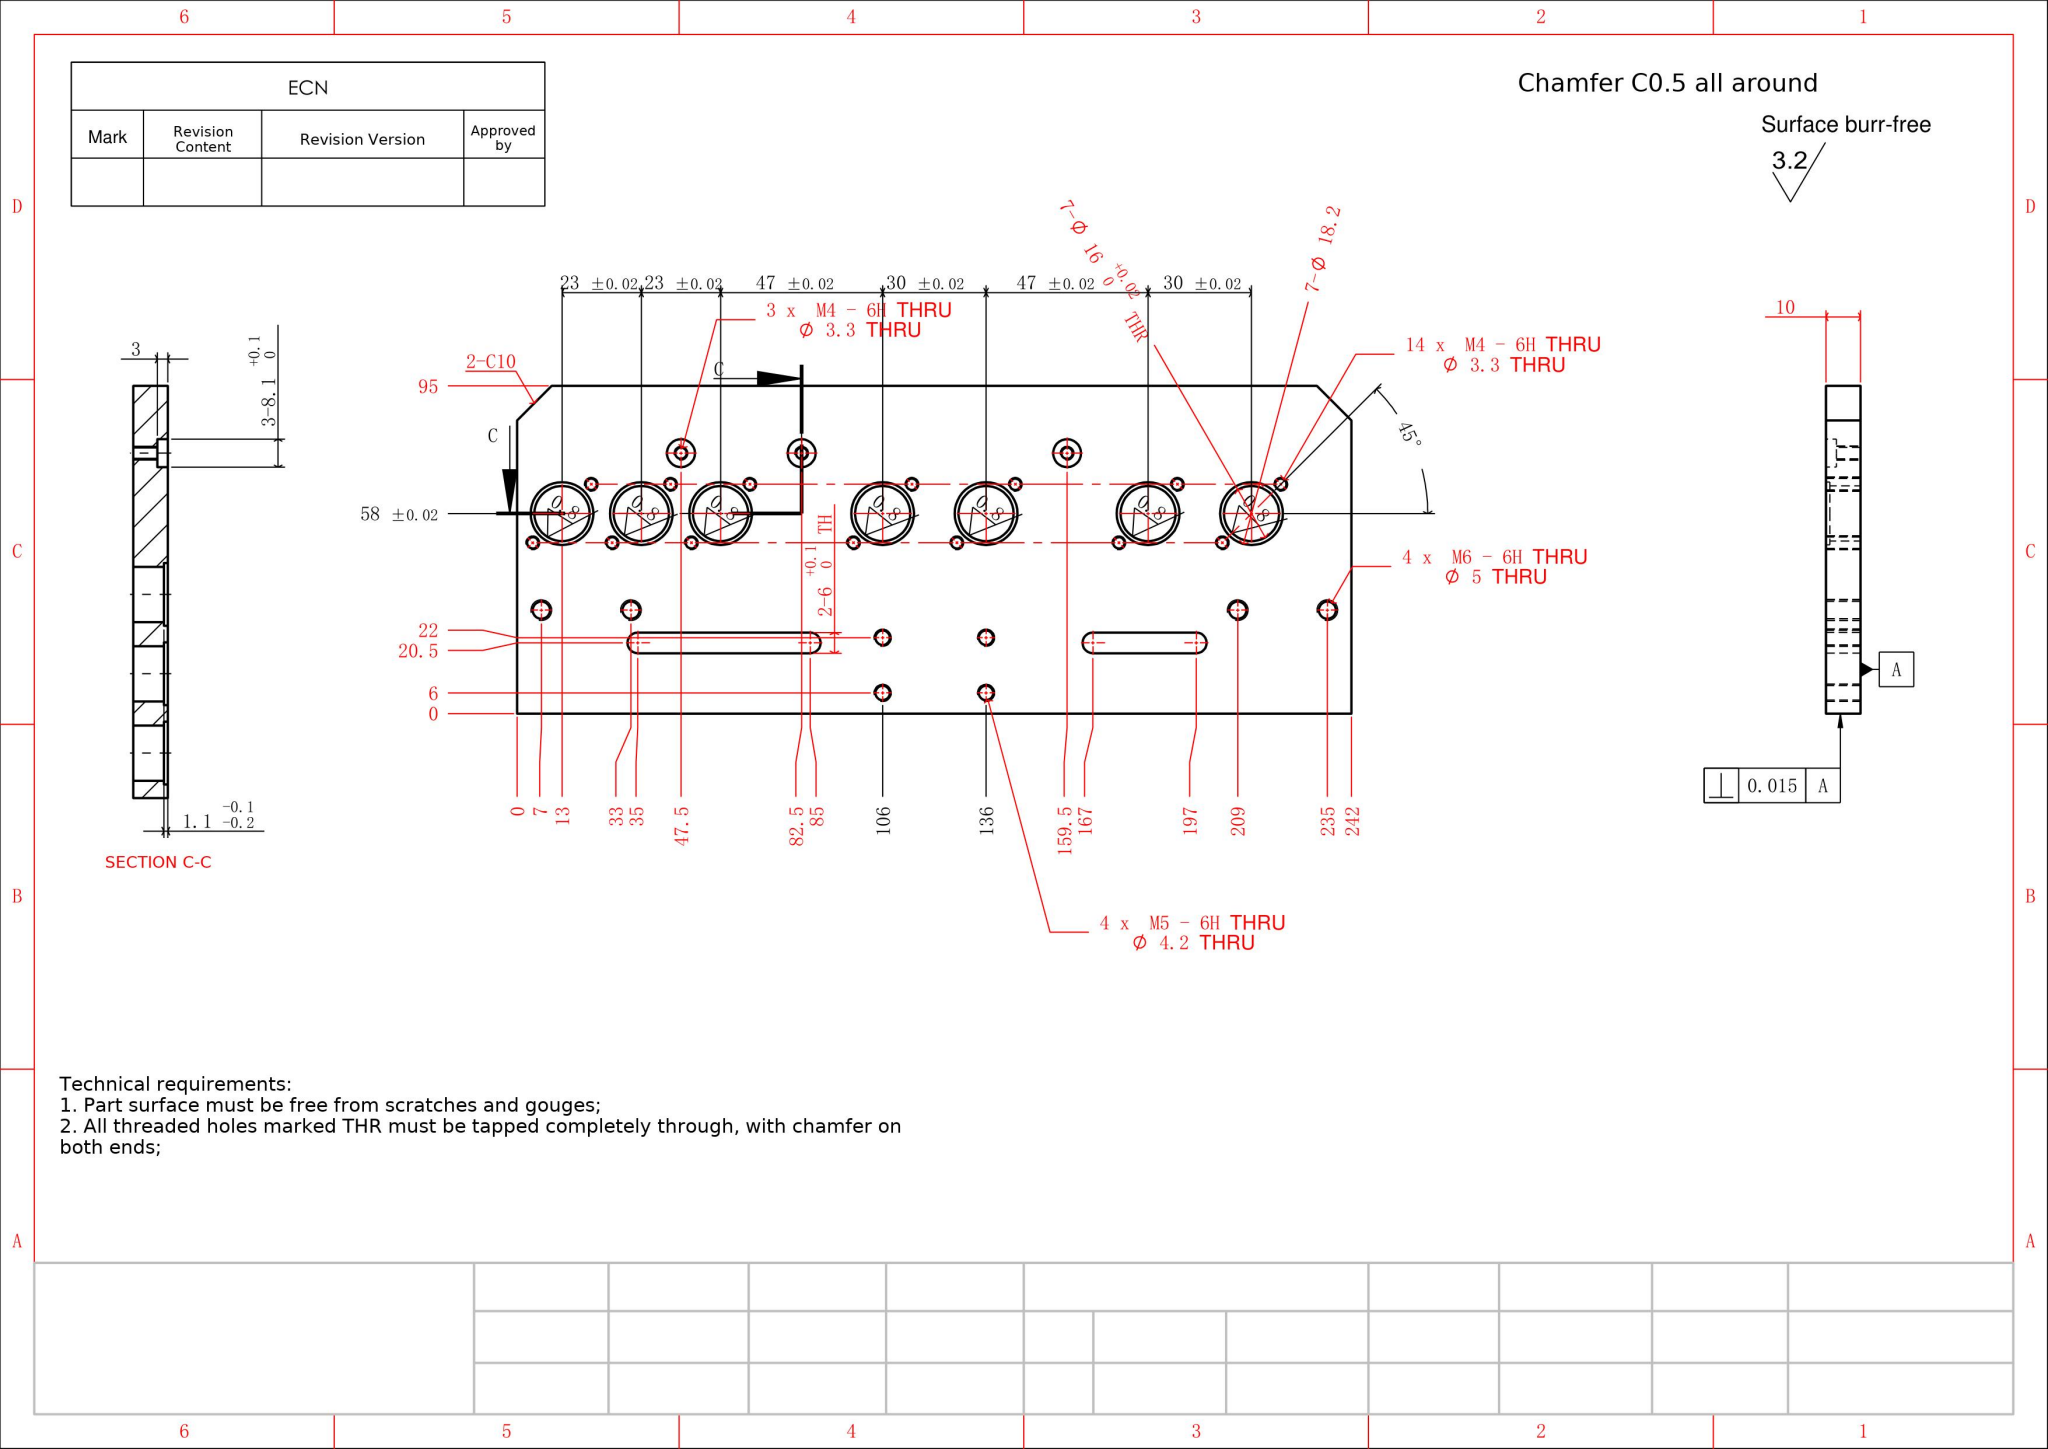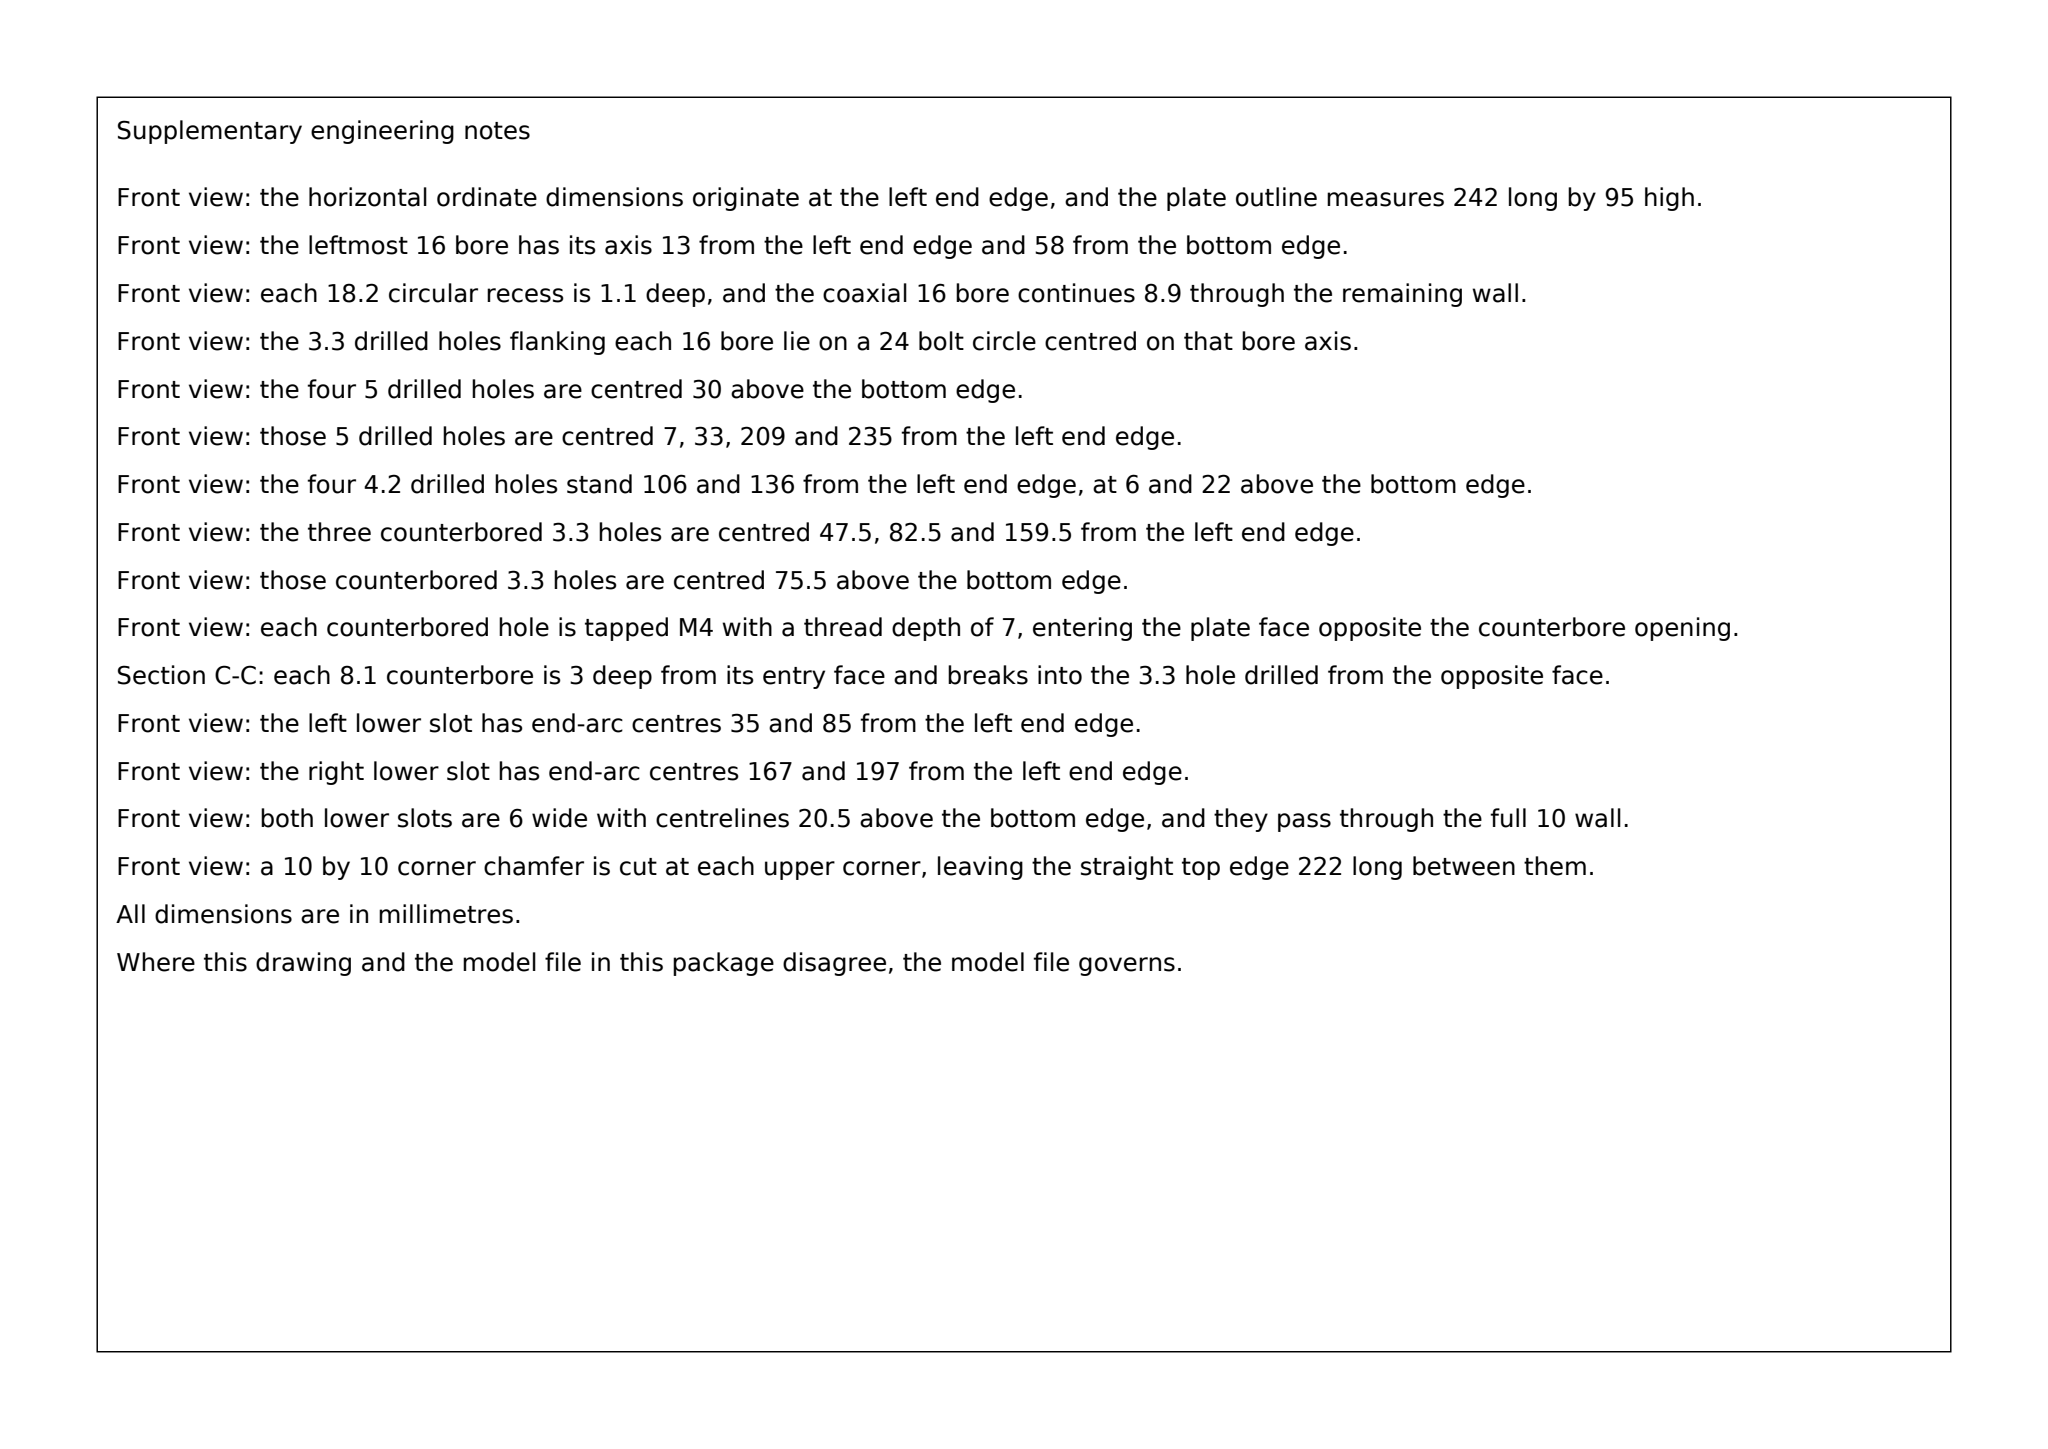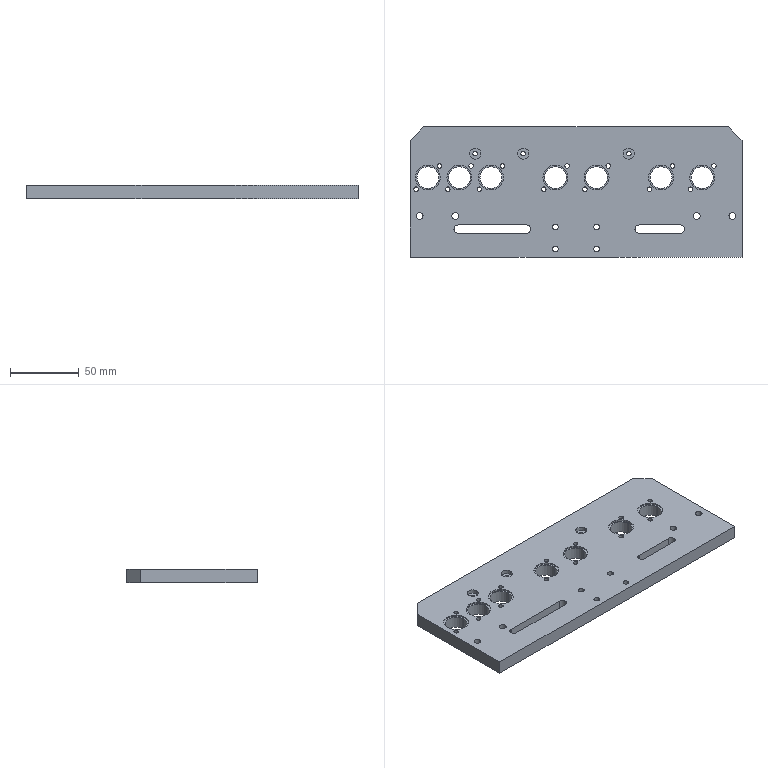Part | SolidWorks | mm | 1 solid | 112 faces | box 242 x 95 x 10 mm | volume 205825 mm3 | cylinder 90 | plane 22 | commonest cylinder face diameters 3.3 x34 18.2 x14 16 x14 4.2 x8 5 x8 6 x6 8.1 x6
Drawing notes:
4x M6-6H THRU (Ø5): CL AT 30 FROM BOTTOM EDGE (Y=0) | from the solid: Ø5.0 thru holes at (7,30),(33,30),(209,30),(235,30); bottom face y=0
2-Ø6 +0.1/0 THRU (SLOT WIDTH, R3 ENDS), SLOT LG 50 & 30 | from the solid: 4 half-cyl Ø6 z0-10 at x35/85 & x167/197, y20.5; walls y17.5-23.5
7-Ø16 +0.02/0 THRU, C'BORE Ø18.2 DP 1.1 FAR SIDE | from the solid: 7 bores Ø16 z0-8.9 @y58; Ø18.2 z8.9-10 same axes
Ø24 B.C.: 14-M4-6H THRU (Ø3.3), 2 PER Ø16 BORE, 45° | from the solid: 14 Ø3.3 thru holes at ±8.5,±8.5 from each Ø16 axis = R12 B.C.
ORD 75.5 = CL OF 3-Ø3.3 HOLES FROM BOT EDGE Y0 (NOT 22) | from the solid: Ø3.3 z0-7 w/ Ø8.1 z7-10 at (47.5,75.5)(82.5,75.5)(159.5,75.5)